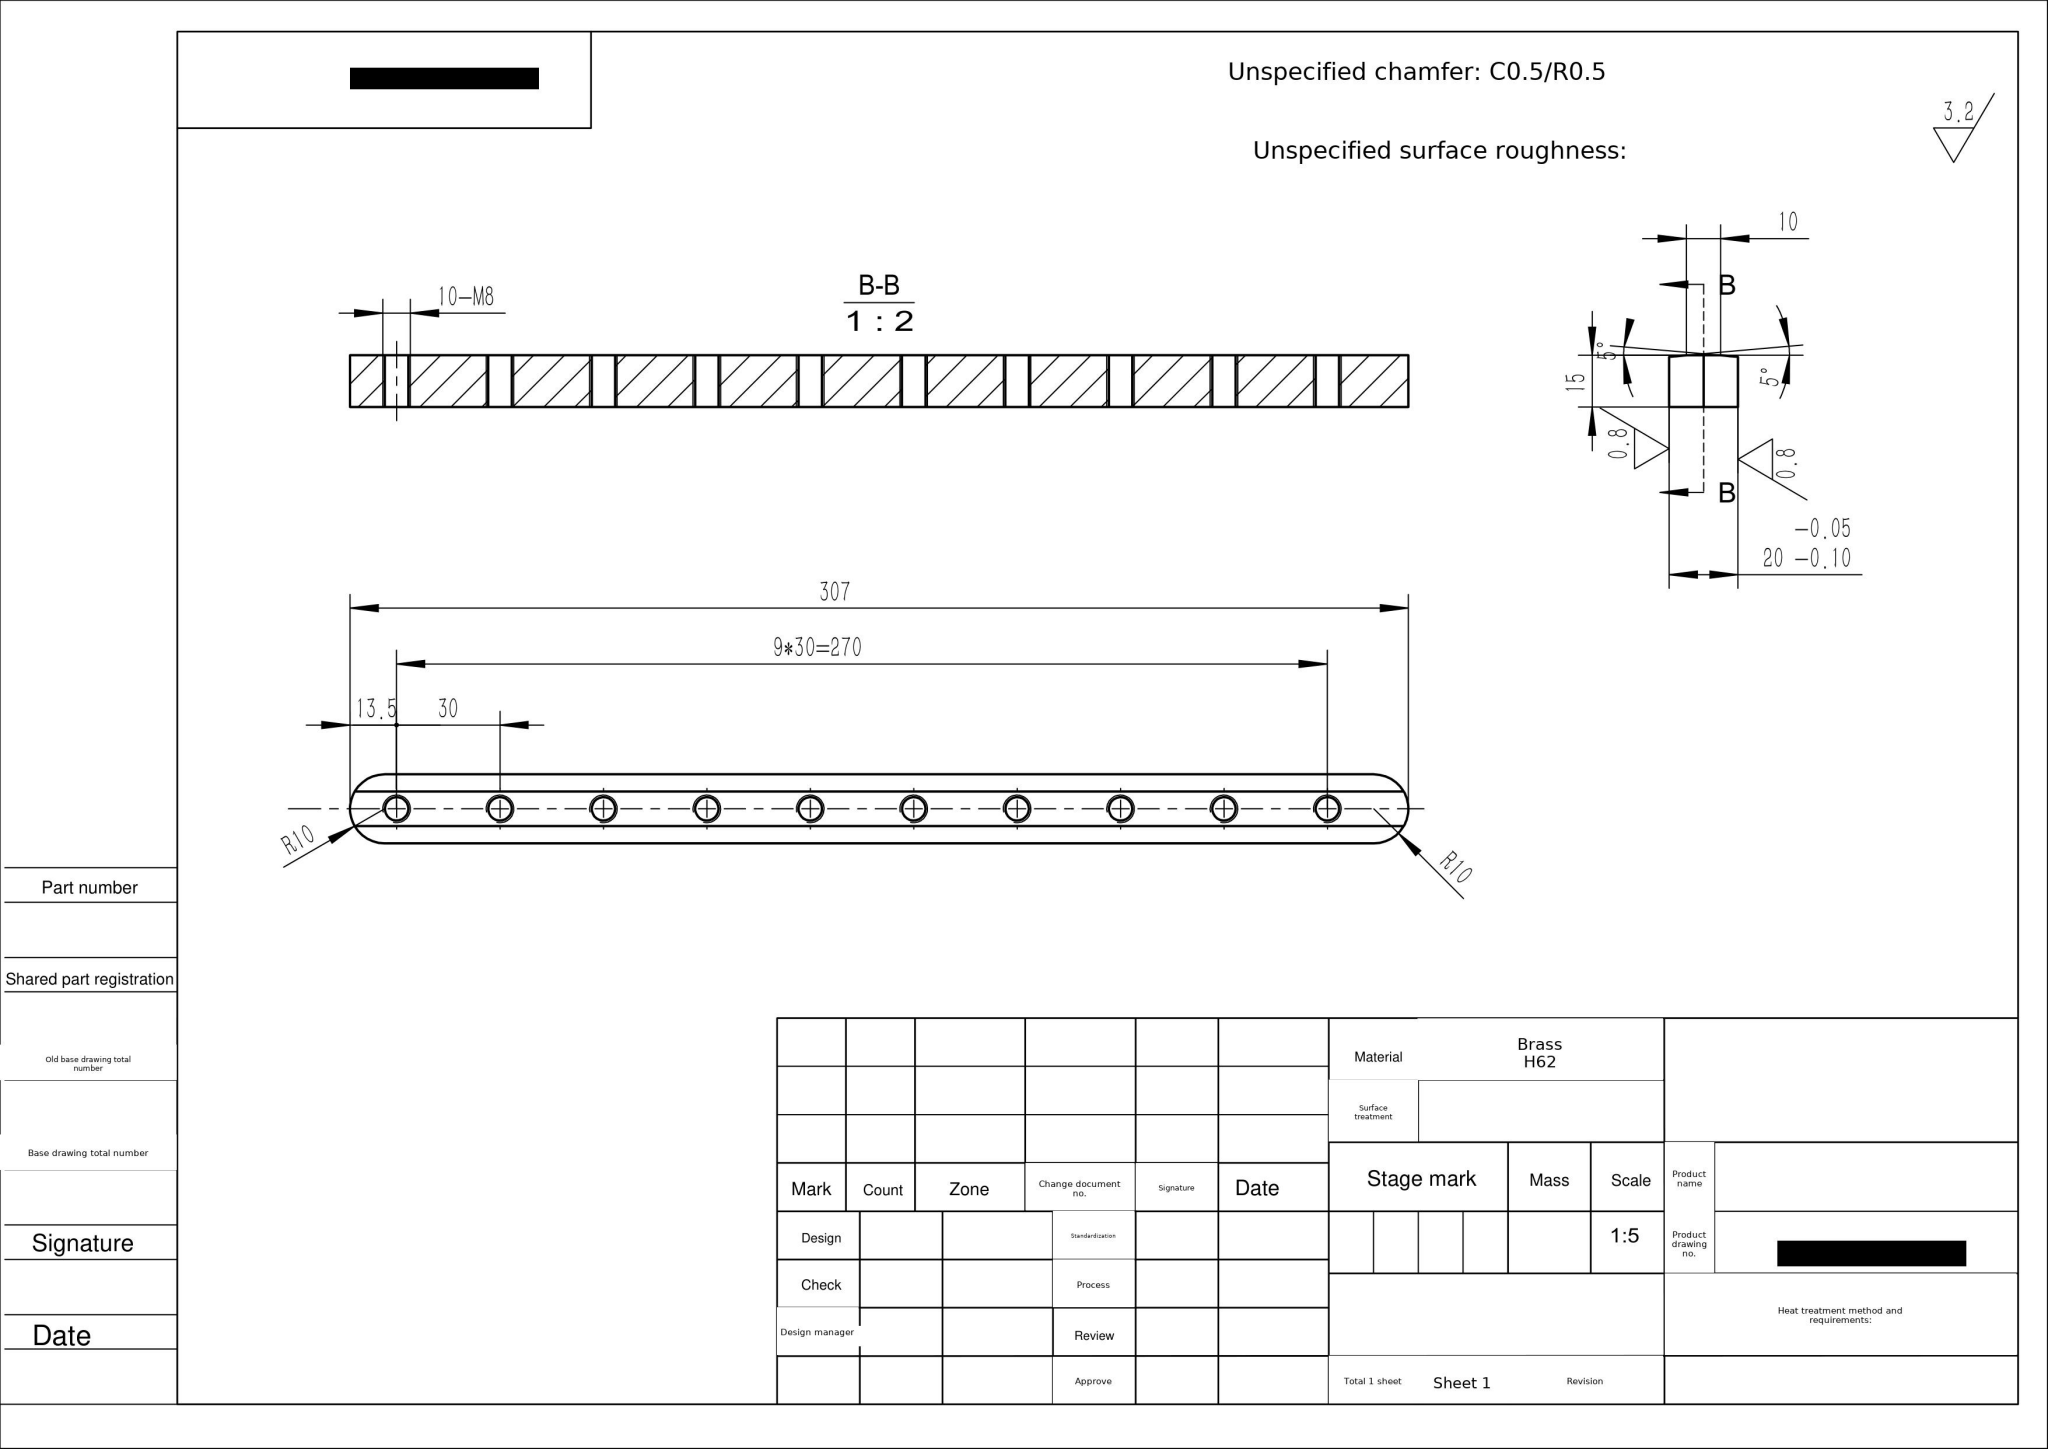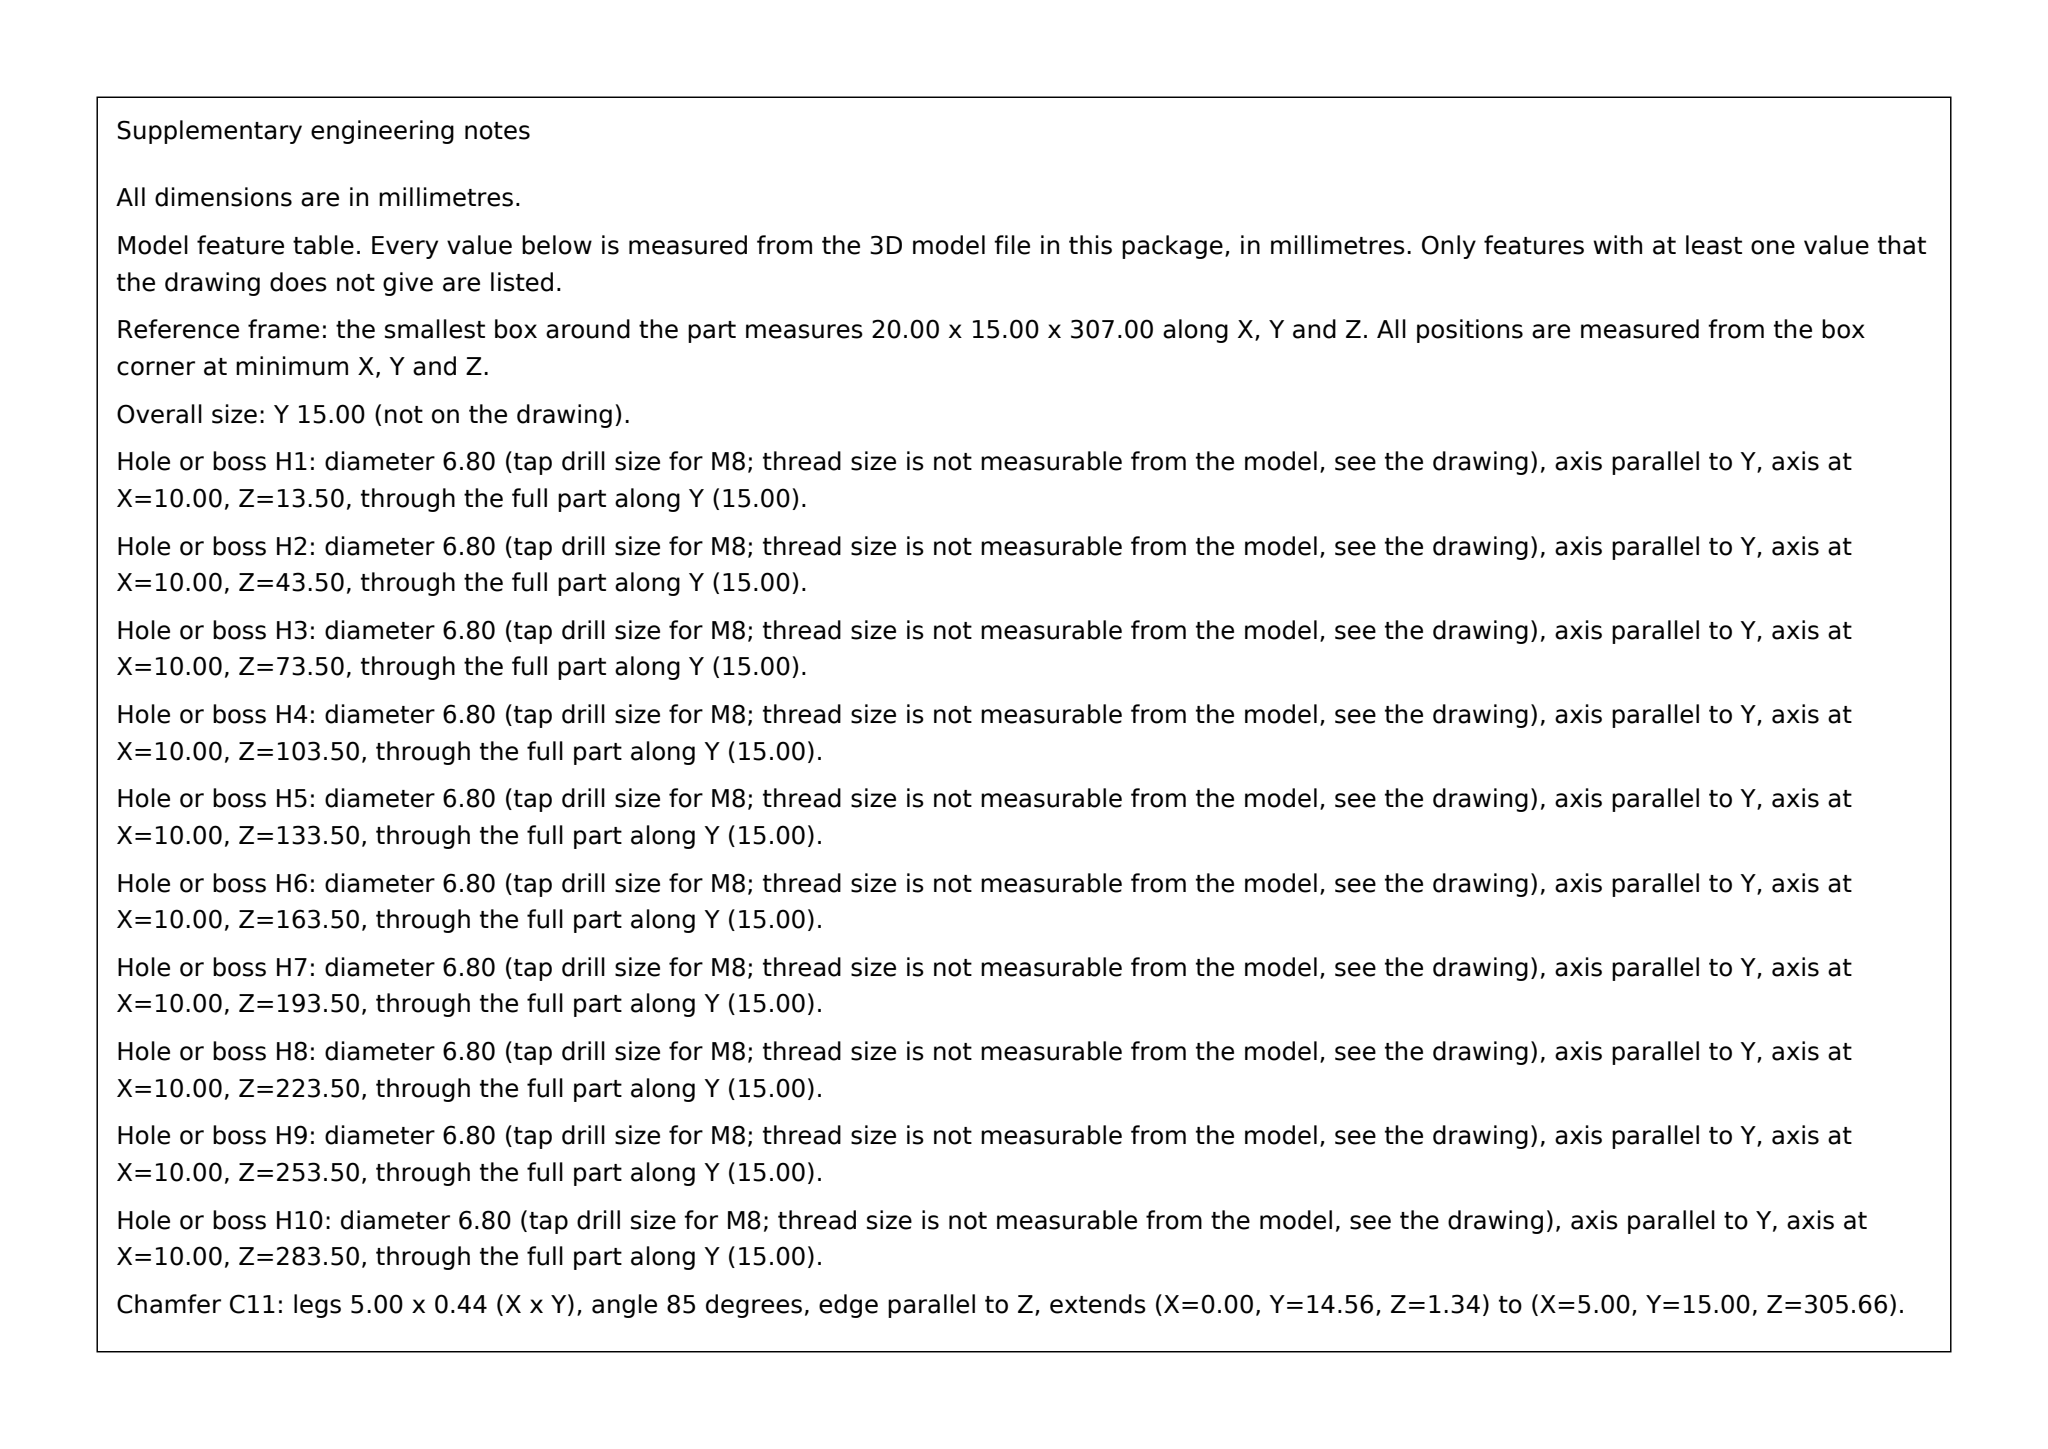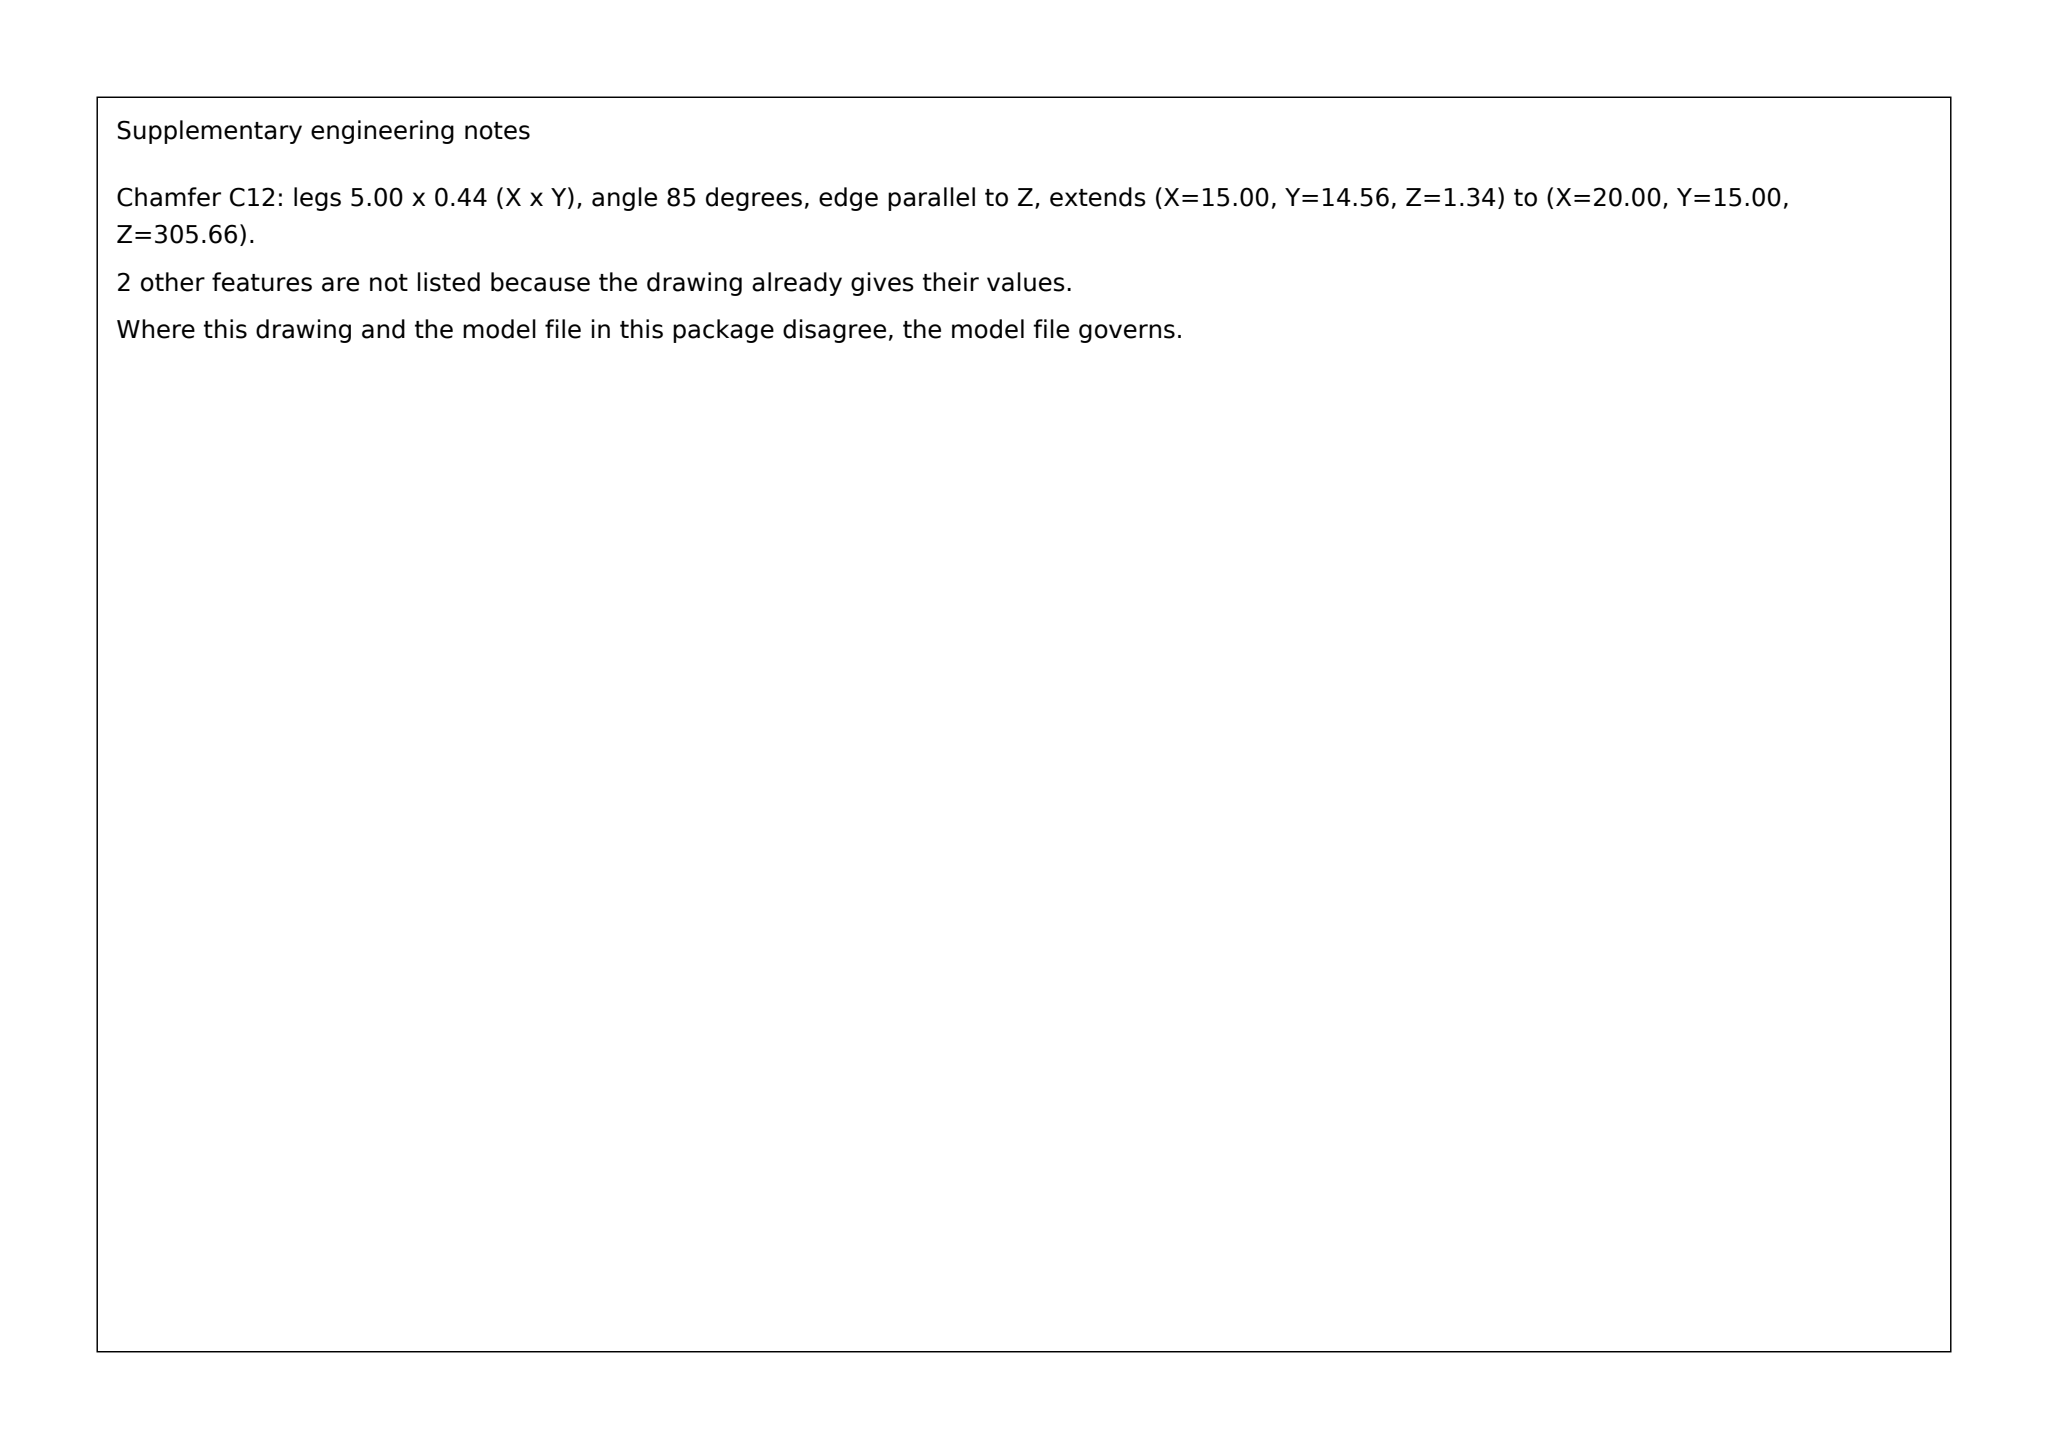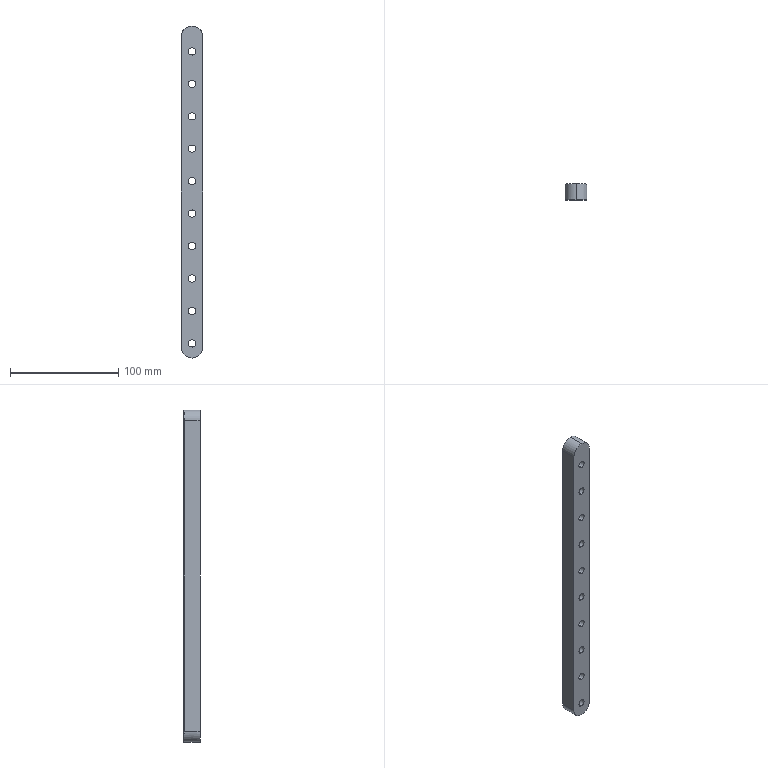Part | SolidWorks | mm | material Brass H62 | 1 solid | 30 faces | box 20 x 15 x 307 mm | volume 84715 mm3 | cylinder 24 | plane 6 | commonest cylinder face diameters 6.8 x20 20 x4